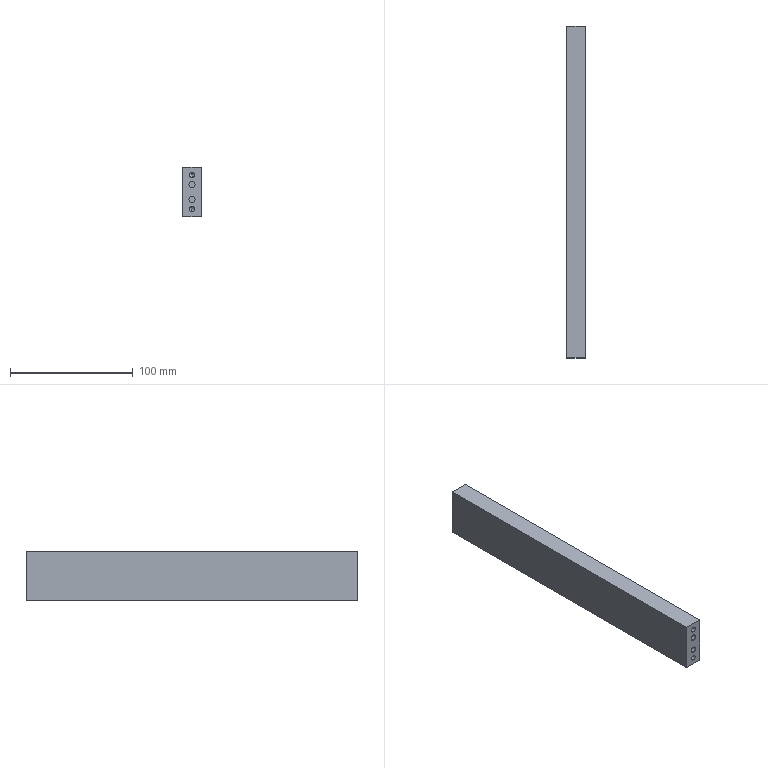Component | SolidWorks | PressingMechanism-12-2 | 1 solid | 34 faces | box 15 x 270 x 40 mm | volume 160573 mm3 | cylinder 16 | plane 10 | cone 8 | commonest cylinder face diameters 5 x8 4.2 x8
build123d program:
from build123d import *

# Parameters (mm, degrees)
SKETCH1_W             = 270
SKETCH1_H             = 40
EXTRUDE1_DEPTH        = 7.5
M5_TAPPED_HOLE1_D     = 4.2
M5_TAPPED_HOLE1_DEPTH = 14
M5_TAPPED_HOLE1_TIP   = 1.262
M5_TAPPED_HOLE2_D     = 4.2
M5_TAPPED_HOLE2_DEPTH = 14
M5_TAPPED_HOLE2_TIP   = 1.262
HOLEWZD1_D            = 5
HOLEWZD1_DEPTH        = 8
HOLEWZD2_D            = 5
HOLEWZD2_DEPTH        = 8


with BuildPart() as part:
    # Sketch1 → Extrude1 (new, symmetric)
    with BuildSketch(Plane(origin=(0, 0, 0), x_dir=(1, 0, 0), z_dir=(0, 1, 0))):
        Rectangle(SKETCH1_W, SKETCH1_H)
    extrude(amount=EXTRUDE1_DEPTH, both=True)

    # M5 Tapped Hole1
    with Locations(Plane(origin=(135, 0, 0), x_dir=(0, 0, -1), z_dir=(1, 0, 0))):
        with Locations((14, 0), (-14, 0)):
            Hole(M5_TAPPED_HOLE1_D / 2, depth=M5_TAPPED_HOLE1_DEPTH)
            with Locations((0, 0, -(M5_TAPPED_HOLE1_DEPTH + M5_TAPPED_HOLE1_TIP / 2))):  # 118° drill point
                Cone(0, M5_TAPPED_HOLE1_D / 2, M5_TAPPED_HOLE1_TIP, mode=Mode.SUBTRACT)

    # M5 Tapped Hole2
    with Locations(Plane.ZY.offset(135)):
        with Locations((-14, 0), (14, 0)):
            Hole(M5_TAPPED_HOLE2_D / 2, depth=M5_TAPPED_HOLE2_DEPTH)
            with Locations((0, 0, -(M5_TAPPED_HOLE2_DEPTH + M5_TAPPED_HOLE2_TIP / 2))):  # 118° drill point
                Cone(0, M5_TAPPED_HOLE2_D / 2, M5_TAPPED_HOLE2_TIP, mode=Mode.SUBTRACT)

    # HoleWzd1
    with Locations(Plane(origin=(135, 0, 0), x_dir=(0, 0, -1), z_dir=(1, 0, 0))):
        with Locations((6, 0), (-6, 0)):
            Hole(HOLEWZD1_D / 2, depth=HOLEWZD1_DEPTH)

    # HoleWzd2
    with Locations(Plane.ZY.offset(135)):
        with Locations((-6, 0), (6, 0)):
            Hole(HOLEWZD2_D / 2, depth=HOLEWZD2_DEPTH)


solid = part.part

# Placed as in the assembly
solid = solid.moved(Location((-192.5, -90, 77), (0, 0, 90)))
STEP:
#1=CARTESIAN_POINT('',(-7.579,-8.543,3.366));
#2=VERTEX_POINT('',#1);
#3=CARTESIAN_POINT('',(-7.579,-8.543,3.169));
#4=VERTEX_POINT('',#3);
#5=CARTESIAN_POINT('',(-7.579,-8.543,3.268));
#6=DIRECTION('',(0.,-1.,0.));
#7=DIRECTION('',(0.,0.,-1.));
#8=AXIS2_PLACEMENT_3D('',#5,#6,#7);
#9=CIRCLE('',#8,0.09843);
#10=EDGE_CURVE('',#2,#4,#9,.T.);
#11=ORIENTED_EDGE('',*,*,#10,.F.);
#12=CARTESIAN_POINT('',(-7.579,-8.858,3.366));
#13=VERTEX_POINT('',#12);
#14=CARTESIAN_POINT('',(-7.579,-8.858,3.366));
#15=DIRECTION('',(0.,-1.,0.));
#16=VECTOR('',#15,39.37);
#17=LINE('',#14,#16);
#18=EDGE_CURVE('',#2,#13,#17,.T.);
#19=ORIENTED_EDGE('',*,*,#18,.T.);
#20=CARTESIAN_POINT('',(-7.579,-8.858,3.169));
#21=VERTEX_POINT('',#20);
#22=CARTESIAN_POINT('',(-7.579,-8.858,3.268));
#23=DIRECTION('',(0.,-1.,0.));
#24=DIRECTION('',(0.,0.,-1.));
#25=AXIS2_PLACEMENT_3D('',#22,#23,#24);
#26=CIRCLE('',#25,0.09843);
#27=EDGE_CURVE('',#13,#21,#26,.T.);
#28=ORIENTED_EDGE('',*,*,#27,.T.);
#29=CARTESIAN_POINT('',(-7.579,-8.858,3.169));
#30=DIRECTION('',(0.,-1.,0.));
#31=VECTOR('',#30,39.37);
#32=LINE('',#29,#31);
#33=EDGE_CURVE('',#4,#21,#32,.T.);
#34=ORIENTED_EDGE('',*,*,#33,.F.);
#35=EDGE_LOOP('',(#11,#19,#28,#34));
#36=FACE_OUTER_BOUND('',#35,.T.);
#37=CARTESIAN_POINT('',(-7.579,-8.858,3.268));
#38=DIRECTION('',(0.,-1.,0.));
#39=DIRECTION('',(0.,0.,-1.));
#40=AXIS2_PLACEMENT_3D('',#37,#38,#39);
#41=CYLINDRICAL_SURFACE('',#40,0.09843);
#42=ADVANCED_FACE('',(#36),#41,.F.);
#43=CARTESIAN_POINT('',(-7.579,-8.543,2.894));
#44=VERTEX_POINT('',#43);
#45=CARTESIAN_POINT('',(-7.579,-8.543,2.697));
#46=VERTEX_POINT('',#45);
#47=CARTESIAN_POINT('',(-7.579,-8.543,2.795));
#48=DIRECTION('',(0.,-1.,0.));
#49=DIRECTION('',(0.,0.,-1.));
#50=AXIS2_PLACEMENT_3D('',#47,#48,#49);
#51=CIRCLE('',#50,0.09843);
#52=EDGE_CURVE('',#44,#46,#51,.T.);
#53=ORIENTED_EDGE('',*,*,#52,.F.);
#54=CARTESIAN_POINT('',(-7.579,-8.858,2.894));
#55=VERTEX_POINT('',#54);
#56=CARTESIAN_POINT('',(-7.579,-8.858,2.894));
#57=DIRECTION('',(0.,-1.,0.));
#58=VECTOR('',#57,39.37);
#59=LINE('',#56,#58);
#60=EDGE_CURVE('',#44,#55,#59,.T.);
#61=ORIENTED_EDGE('',*,*,#60,.T.);
#62=CARTESIAN_POINT('',(-7.579,-8.858,2.697));
#63=VERTEX_POINT('',#62);
#64=CARTESIAN_POINT('',(-7.579,-8.858,2.795));
#65=DIRECTION('',(0.,-1.,0.));
#66=DIRECTION('',(0.,0.,-1.));
#67=AXIS2_PLACEMENT_3D('',#64,#65,#66);
#68=CIRCLE('',#67,0.09843);
#69=EDGE_CURVE('',#55,#63,#68,.T.);
#70=ORIENTED_EDGE('',*,*,#69,.T.);
#71=CARTESIAN_POINT('',(-7.579,-8.858,2.697));
#72=DIRECTION('',(0.,-1.,0.));
#73=VECTOR('',#72,39.37);
#74=LINE('',#71,#73);
#75=EDGE_CURVE('',#46,#63,#74,.T.);
#76=ORIENTED_EDGE('',*,*,#75,.F.);
#77=EDGE_LOOP('',(#53,#61,#70,#76));
#78=FACE_OUTER_BOUND('',#77,.T.);
#79=CARTESIAN_POINT('',(-7.579,-8.858,2.795));
#80=DIRECTION('',(0.,-1.,0.));
#81=DIRECTION('',(0.,0.,-1.));
#82=AXIS2_PLACEMENT_3D('',#79,#80,#81);
#83=CYLINDRICAL_SURFACE('',#82,0.09843);
#84=ADVANCED_FACE('',(#78),#83,.F.);
#85=CARTESIAN_POINT('',(-7.579,1.457,3.169));
#86=VERTEX_POINT('',#85);
#87=CARTESIAN_POINT('',(-7.579,1.457,3.366));
#88=VERTEX_POINT('',#87);
#89=CARTESIAN_POINT('',(-7.579,1.457,3.268));
#90=DIRECTION('',(-0.,1.,-0.));
#91=DIRECTION('',(0.,0.,1.));
#92=AXIS2_PLACEMENT_3D('',#89,#90,#91);
#93=CIRCLE('',#92,0.09843);
#94=EDGE_CURVE('',#86,#88,#93,.T.);
#95=ORIENTED_EDGE('',*,*,#94,.F.);
#96=CARTESIAN_POINT('',(-7.579,1.772,3.169));
#97=VERTEX_POINT('',#96);
#98=CARTESIAN_POINT('',(-7.579,1.772,3.169));
#99=DIRECTION('',(-0.,1.,-0.));
#100=VECTOR('',#99,39.37);
#101=LINE('',#98,#100);
#102=EDGE_CURVE('',#86,#97,#101,.T.);
#103=ORIENTED_EDGE('',*,*,#102,.T.);
#104=CARTESIAN_POINT('',(-7.579,1.772,3.366));
#105=VERTEX_POINT('',#104);
#106=CARTESIAN_POINT('',(-7.579,1.772,3.268));
#107=DIRECTION('',(-0.,1.,-0.));
#108=DIRECTION('',(0.,0.,1.));
#109=AXIS2_PLACEMENT_3D('',#106,#107,#108);
#110=CIRCLE('',#109,0.09843);
#111=EDGE_CURVE('',#97,#105,#110,.T.);
#112=ORIENTED_EDGE('',*,*,#111,.T.);
#113=CARTESIAN_POINT('',(-7.579,1.772,3.366));
#114=DIRECTION('',(-0.,1.,-0.));
#115=VECTOR('',#114,39.37);
#116=LINE('',#113,#115);
#117=EDGE_CURVE('',#88,#105,#116,.T.);
#118=ORIENTED_EDGE('',*,*,#117,.F.);
#119=EDGE_LOOP('',(#95,#103,#112,#118));
#120=FACE_OUTER_BOUND('',#119,.T.);
#121=CARTESIAN_POINT('',(-7.579,1.772,3.268));
#122=DIRECTION('',(-0.,1.,-0.));
#123=DIRECTION('',(0.,0.,1.));
#124=AXIS2_PLACEMENT_3D('',#121,#122,#123);
#125=CYLINDRICAL_SURFACE('',#124,0.09843);
#126=ADVANCED_FACE('',(#120),#125,.F.);
#127=CARTESIAN_POINT('',(-7.579,1.457,2.697));
#128=VERTEX_POINT('',#127);
#129=CARTESIAN_POINT('',(-7.579,1.457,2.894));
#130=VERTEX_POINT('',#129);
#131=CARTESIAN_POINT('',(-7.579,1.457,2.795));
#132=DIRECTION('',(-0.,1.,-0.));
#133=DIRECTION('',(0.,0.,1.));
#134=AXIS2_PLACEMENT_3D('',#131,#132,#133);
#135=CIRCLE('',#134,0.09843);
#136=EDGE_CURVE('',#128,#130,#135,.T.);
#137=ORIENTED_EDGE('',*,*,#136,.F.);
#138=CARTESIAN_POINT('',(-7.579,1.772,2.697));
#139=VERTEX_POINT('',#138);
#140=CARTESIAN_POINT('',(-7.579,1.772,2.697));
#141=DIRECTION('',(-0.,1.,-0.));
#142=VECTOR('',#141,39.37);
#143=LINE('',#140,#142);
#144=EDGE_CURVE('',#128,#139,#143,.T.);
#145=ORIENTED_EDGE('',*,*,#144,.T.);
#146=CARTESIAN_POINT('',(-7.579,1.772,2.894));
#147=VERTEX_POINT('',#146);
#148=CARTESIAN_POINT('',(-7.579,1.772,2.795));
#149=DIRECTION('',(-0.,1.,-0.));
#150=DIRECTION('',(0.,0.,1.));
#151=AXIS2_PLACEMENT_3D('',#148,#149,#150);
#152=CIRCLE('',#151,0.09843);
#153=EDGE_CURVE('',#139,#147,#152,.T.);
#154=ORIENTED_EDGE('',*,*,#153,.T.);
#155=CARTESIAN_POINT('',(-7.579,1.772,2.894));
#156=DIRECTION('',(-0.,1.,-0.));
#157=VECTOR('',#156,39.37);
#158=LINE('',#155,#157);
#159=EDGE_CURVE('',#130,#147,#158,.T.);
#160=ORIENTED_EDGE('',*,*,#159,.F.);
#161=EDGE_LOOP('',(#137,#145,#154,#160));
#162=FACE_OUTER_BOUND('',#161,.T.);
#163=CARTESIAN_POINT('',(-7.579,1.772,2.795));
#164=DIRECTION('',(-0.,1.,-0.));
#165=DIRECTION('',(0.,0.,1.));
#166=AXIS2_PLACEMENT_3D('',#163,#164,#165);
#167=CYLINDRICAL_SURFACE('',#166,0.09843);
#168=ADVANCED_FACE('',(#162),#167,.F.);
#169=CARTESIAN_POINT('',(-7.579,-8.307,3.665));
#170=VERTEX_POINT('',#169);
#171=CARTESIAN_POINT('',(-7.579,-8.307,3.5));
#172=VERTEX_POINT('',#171);
#173=CARTESIAN_POINT('',(-7.579,-8.307,3.583));
#174=DIRECTION('',(0.,-1.,0.));
#175=DIRECTION('',(0.,0.,-1.));
#176=AXIS2_PLACEMENT_3D('',#173,#174,#175);
#177=CIRCLE('',#176,0.08268);
#178=EDGE_CURVE('',#170,#172,#177,.T.);
#179=ORIENTED_EDGE('',*,*,#178,.F.);
#180=CARTESIAN_POINT('',(-7.579,-8.858,3.665));
#181=VERTEX_POINT('',#180);
#182=CARTESIAN_POINT('',(-7.579,-8.858,3.665));
#183=DIRECTION('',(0.,-1.,0.));
#184=VECTOR('',#183,39.37);
#185=LINE('',#182,#184);
#186=EDGE_CURVE('',#170,#181,#185,.T.);
#187=ORIENTED_EDGE('',*,*,#186,.T.);
#188=CARTESIAN_POINT('',(-7.579,-8.858,3.5));
#189=VERTEX_POINT('',#188);
#190=CARTESIAN_POINT('',(-7.579,-8.858,3.583));
#191=DIRECTION('',(0.,-1.,0.));
#192=DIRECTION('',(0.,0.,-1.));
#193=AXIS2_PLACEMENT_3D('',#190,#191,#192);
#194=CIRCLE('',#193,0.08268);
#195=EDGE_CURVE('',#181,#189,#194,.T.);
#196=ORIENTED_EDGE('',*,*,#195,.T.);
#197=CARTESIAN_POINT('',(-7.579,-8.858,3.5));
#198=DIRECTION('',(0.,-1.,0.));
#199=VECTOR('',#198,39.37);
#200=LINE('',#197,#199);
#201=EDGE_CURVE('',#172,#189,#200,.T.);
#202=ORIENTED_EDGE('',*,*,#201,.F.);
#203=EDGE_LOOP('',(#179,#187,#196,#202));
#204=FACE_OUTER_BOUND('',#203,.T.);
#205=CARTESIAN_POINT('',(-7.579,-8.858,3.583));
#206=DIRECTION('',(0.,-1.,0.));
#207=DIRECTION('',(0.,0.,-1.));
#208=AXIS2_PLACEMENT_3D('',#205,#206,#207);
#209=CYLINDRICAL_SURFACE('',#208,0.08268);
#210=ADVANCED_FACE('',(#204),#209,.F.);
#211=CARTESIAN_POINT('',(-7.579,-8.257,3.583));
#212=VERTEX_POINT('',#211);
#213=CARTESIAN_POINT('',(-7.579,-8.307,3.5));
#214=DIRECTION('',(-0.,-0.515,-0.8572));
#215=VECTOR('',#214,39.37);
#216=LINE('',#213,#215);
#217=EDGE_CURVE('',#212,#172,#216,.T.);
#218=ORIENTED_EDGE('',*,*,#217,.F.);
#219=CARTESIAN_POINT('',(-7.579,-8.307,3.665));
#220=DIRECTION('',(0.,-0.515,0.8572));
#221=VECTOR('',#220,39.37);
#222=LINE('',#219,#221);
#223=EDGE_CURVE('',#212,#170,#222,.T.);
#224=ORIENTED_EDGE('',*,*,#223,.T.);
#225=ORIENTED_EDGE('',*,*,#178,.T.);
#226=EDGE_LOOP('',(#218,#224,#225));
#227=FACE_OUTER_BOUND('',#226,.T.);
#228=CARTESIAN_POINT('',(-7.579,-8.307,3.583));
#229=DIRECTION('',(0.,-1.,0.));
#230=DIRECTION('',(0.,0.,-1.));
#231=AXIS2_PLACEMENT_3D('',#228,#229,#230);
#232=CONICAL_SURFACE('',#231,0.08268,1.03);
#233=ADVANCED_FACE('',(#227),#232,.F.);
#234=CARTESIAN_POINT('',(-7.579,-8.307,2.563));
#235=VERTEX_POINT('',#234);
#236=CARTESIAN_POINT('',(-7.579,-8.307,2.398));
#237=VERTEX_POINT('',#236);
#238=CARTESIAN_POINT('',(-7.579,-8.307,2.48));
#239=DIRECTION('',(0.,-1.,0.));
#240=DIRECTION('',(0.,0.,-1.));
#241=AXIS2_PLACEMENT_3D('',#238,#239,#240);
#242=CIRCLE('',#241,0.08268);
#243=EDGE_CURVE('',#235,#237,#242,.T.);
#244=ORIENTED_EDGE('',*,*,#243,.F.);
#245=CARTESIAN_POINT('',(-7.579,-8.858,2.563));
#246=VERTEX_POINT('',#245);
#247=CARTESIAN_POINT('',(-7.579,-8.858,2.563));
#248=DIRECTION('',(0.,-1.,0.));
#249=VECTOR('',#248,39.37);
#250=LINE('',#247,#249);
#251=EDGE_CURVE('',#235,#246,#250,.T.);
#252=ORIENTED_EDGE('',*,*,#251,.T.);
#253=CARTESIAN_POINT('',(-7.579,-8.858,2.398));
#254=VERTEX_POINT('',#253);
#255=CARTESIAN_POINT('',(-7.579,-8.858,2.48));
#256=DIRECTION('',(0.,-1.,0.));
#257=DIRECTION('',(0.,0.,-1.));
#258=AXIS2_PLACEMENT_3D('',#255,#256,#257);
#259=CIRCLE('',#258,0.08268);
#260=EDGE_CURVE('',#246,#254,#259,.T.);
#261=ORIENTED_EDGE('',*,*,#260,.T.);
#262=CARTESIAN_POINT('',(-7.579,-8.858,2.398));
#263=DIRECTION('',(0.,-1.,0.));
#264=VECTOR('',#263,39.37);
#265=LINE('',#262,#264);
#266=EDGE_CURVE('',#237,#254,#265,.T.);
#267=ORIENTED_EDGE('',*,*,#266,.F.);
#268=EDGE_LOOP('',(#244,#252,#261,#267));
#269=FACE_OUTER_BOUND('',#268,.T.);
#270=CARTESIAN_POINT('',(-7.579,-8.858,2.48));
#271=DIRECTION('',(0.,-1.,0.));
#272=DIRECTION('',(0.,0.,-1.));
#273=AXIS2_PLACEMENT_3D('',#270,#271,#272);
#274=CYLINDRICAL_SURFACE('',#273,0.08268);
#275=ADVANCED_FACE('',(#269),#274,.F.);
#276=CARTESIAN_POINT('',(-7.579,-8.257,2.48));
#277=VERTEX_POINT('',#276);
#278=CARTESIAN_POINT('',(-7.579,-8.307,2.398));
#279=DIRECTION('',(-0.,-0.515,-0.8572));
#280=VECTOR('',#279,39.37);
#281=LINE('',#278,#280);
#282=EDGE_CURVE('',#277,#237,#281,.T.);
#283=ORIENTED_EDGE('',*,*,#282,.F.);
#284=CARTESIAN_POINT('',(-7.579,-8.307,2.563));
#285=DIRECTION('',(0.,-0.515,0.8572));
#286=VECTOR('',#285,39.37);
#287=LINE('',#284,#286);
#288=EDGE_CURVE('',#277,#235,#287,.T.);
#289=ORIENTED_EDGE('',*,*,#288,.T.);
#290=ORIENTED_EDGE('',*,*,#243,.T.);
#291=EDGE_LOOP('',(#283,#289,#290));
#292=FACE_OUTER_BOUND('',#291,.T.);
#293=CARTESIAN_POINT('',(-7.579,-8.307,2.48));
#294=DIRECTION('',(0.,-1.,0.));
#295=DIRECTION('',(0.,0.,-1.));
#296=AXIS2_PLACEMENT_3D('',#293,#294,#295);
#297=CONICAL_SURFACE('',#296,0.08268,1.03);
#298=ADVANCED_FACE('',(#292),#297,.F.);
#299=CARTESIAN_POINT('',(-7.579,1.22,3.5));
#300=VERTEX_POINT('',#299);
#301=CARTESIAN_POINT('',(-7.579,1.22,3.665));
#302=VERTEX_POINT('',#301);
#303=CARTESIAN_POINT('',(-7.579,1.22,3.583));
#304=DIRECTION('',(-0.,1.,-0.));
#305=DIRECTION('',(0.,0.,1.));
#306=AXIS2_PLACEMENT_3D('',#303,#304,#305);
#307=CIRCLE('',#306,0.08268);
#308=EDGE_CURVE('',#300,#302,#307,.T.);
#309=ORIENTED_EDGE('',*,*,#308,.F.);
#310=CARTESIAN_POINT('',(-7.579,1.772,3.5));
#311=VERTEX_POINT('',#310);
#312=CARTESIAN_POINT('',(-7.579,1.772,3.5));
#313=DIRECTION('',(-0.,1.,-0.));
#314=VECTOR('',#313,39.37);
#315=LINE('',#312,#314);
#316=EDGE_CURVE('',#300,#311,#315,.T.);
#317=ORIENTED_EDGE('',*,*,#316,.T.);
#318=CARTESIAN_POINT('',(-7.579,1.772,3.665));
#319=VERTEX_POINT('',#318);
#320=CARTESIAN_POINT('',(-7.579,1.772,3.583));
#321=DIRECTION('',(-0.,1.,-0.));
#322=DIRECTION('',(0.,0.,1.));
#323=AXIS2_PLACEMENT_3D('',#320,#321,#322);
#324=CIRCLE('',#323,0.08268);
#325=EDGE_CURVE('',#311,#319,#324,.T.);
#326=ORIENTED_EDGE('',*,*,#325,.T.);
#327=CARTESIAN_POINT('',(-7.579,1.772,3.665));
#328=DIRECTION('',(-0.,1.,-0.));
#329=VECTOR('',#328,39.37);
#330=LINE('',#327,#329);
#331=EDGE_CURVE('',#302,#319,#330,.T.);
#332=ORIENTED_EDGE('',*,*,#331,.F.);
#333=EDGE_LOOP('',(#309,#317,#326,#332));
#334=FACE_OUTER_BOUND('',#333,.T.);
#335=CARTESIAN_POINT('',(-7.579,1.772,3.583));
#336=DIRECTION('',(-0.,1.,-0.));
#337=DIRECTION('',(0.,0.,1.));
#338=AXIS2_PLACEMENT_3D('',#335,#336,#337);
#339=CYLINDRICAL_SURFACE('',#338,0.08268);
#340=ADVANCED_FACE('',(#334),#339,.F.);
#341=CARTESIAN_POINT('',(-7.579,1.171,3.583));
#342=VERTEX_POINT('',#341);
#343=CARTESIAN_POINT('',(-7.579,1.22,3.665));
#344=DIRECTION('',(0.,0.515,0.8572));
#345=VECTOR('',#344,39.37);
#346=LINE('',#343,#345);
#347=EDGE_CURVE('',#342,#302,#346,.T.);
#348=ORIENTED_EDGE('',*,*,#347,.F.);
#349=CARTESIAN_POINT('',(-7.579,1.22,3.5));
#350=DIRECTION('',(-0.,0.515,-0.8572));
#351=VECTOR('',#350,39.37);
#352=LINE('',#349,#351);
#353=EDGE_CURVE('',#342,#300,#352,.T.);
#354=ORIENTED_EDGE('',*,*,#353,.T.);
#355=ORIENTED_EDGE('',*,*,#308,.T.);
#356=EDGE_LOOP('',(#348,#354,#355));
#357=FACE_OUTER_BOUND('',#356,.T.);
#358=CARTESIAN_POINT('',(-7.579,1.22,3.583));
#359=DIRECTION('',(-0.,1.,-0.));
#360=DIRECTION('',(0.,0.,1.));
#361=AXIS2_PLACEMENT_3D('',#358,#359,#360);
#362=CONICAL_SURFACE('',#361,0.08268,1.03);
#363=ADVANCED_FACE('',(#357),#362,.F.);
#364=CARTESIAN_POINT('',(-7.579,1.22,2.398));
#365=VERTEX_POINT('',#364);
#366=CARTESIAN_POINT('',(-7.579,1.22,2.563));
#367=VERTEX_POINT('',#366);
#368=CARTESIAN_POINT('',(-7.579,1.22,2.48));
#369=DIRECTION('',(-0.,1.,-0.));
#370=DIRECTION('',(0.,0.,1.));
#371=AXIS2_PLACEMENT_3D('',#368,#369,#370);
#372=CIRCLE('',#371,0.08268);
#373=EDGE_CURVE('',#365,#367,#372,.T.);
#374=ORIENTED_EDGE('',*,*,#373,.F.);
#375=CARTESIAN_POINT('',(-7.579,1.772,2.398));
#376=VERTEX_POINT('',#375);
#377=CARTESIAN_POINT('',(-7.579,1.772,2.398));
#378=DIRECTION('',(-0.,1.,-0.));
#379=VECTOR('',#378,39.37);
#380=LINE('',#377,#379);
#381=EDGE_CURVE('',#365,#376,#380,.T.);
#382=ORIENTED_EDGE('',*,*,#381,.T.);
#383=CARTESIAN_POINT('',(-7.579,1.772,2.563));
#384=VERTEX_POINT('',#383);
#385=CARTESIAN_POINT('',(-7.579,1.772,2.48));
#386=DIRECTION('',(-0.,1.,-0.));
#387=DIRECTION('',(0.,0.,1.));
#388=AXIS2_PLACEMENT_3D('',#385,#386,#387);
#389=CIRCLE('',#388,0.08268);
#390=EDGE_CURVE('',#376,#384,#389,.T.);
#391=ORIENTED_EDGE('',*,*,#390,.T.);
#392=CARTESIAN_POINT('',(-7.579,1.772,2.563));
#393=DIRECTION('',(-0.,1.,-0.));
#394=VECTOR('',#393,39.37);
#395=LINE('',#392,#394);
#396=EDGE_CURVE('',#367,#384,#395,.T.);
#397=ORIENTED_EDGE('',*,*,#396,.F.);
#398=EDGE_LOOP('',(#374,#382,#391,#397));
#399=FACE_OUTER_BOUND('',#398,.T.);
#400=CARTESIAN_POINT('',(-7.579,1.772,2.48));
#401=DIRECTION('',(-0.,1.,-0.));
#402=DIRECTION('',(0.,0.,1.));
#403=AXIS2_PLACEMENT_3D('',#400,#401,#402);
#404=CYLINDRICAL_SURFACE('',#403,0.08268);
#405=ADVANCED_FACE('',(#399),#404,.F.);
#406=CARTESIAN_POINT('',(-7.579,1.171,2.48));
#407=VERTEX_POINT('',#406);
#408=CARTESIAN_POINT('',(-7.579,1.22,2.563));
#409=DIRECTION('',(0.,0.515,0.8572));
#410=VECTOR('',#409,39.37);
#411=LINE('',#408,#410);
#412=EDGE_CURVE('',#407,#367,#411,.T.);
#413=ORIENTED_EDGE('',*,*,#412,.F.);
#414=CARTESIAN_POINT('',(-7.579,1.22,2.398));
#415=DIRECTION('',(-0.,0.515,-0.8572));
#416=VECTOR('',#415,39.37);
#417=LINE('',#414,#416);
#418=EDGE_CURVE('',#407,#365,#417,.T.);
#419=ORIENTED_EDGE('',*,*,#418,.T.);
#420=ORIENTED_EDGE('',*,*,#373,.T.);
#421=EDGE_LOOP('',(#413,#419,#420));
#422=FACE_OUTER_BOUND('',#421,.T.);
#423=CARTESIAN_POINT('',(-7.579,1.22,2.48));
#424=DIRECTION('',(-0.,1.,-0.));
#425=DIRECTION('',(0.,0.,1.));
#426=AXIS2_PLACEMENT_3D('',#423,#424,#425);
#427=CONICAL_SURFACE('',#426,0.08268,1.03);
#428=ADVANCED_FACE('',(#422),#427,.F.);
#429=CARTESIAN_POINT('',(-7.579,-8.858,3.268));
#430=DIRECTION('',(0.,-1.,0.));
#431=DIRECTION('',(0.,0.,-1.));
#432=AXIS2_PLACEMENT_3D('',#429,#430,#431);
#433=CIRCLE('',#432,0.09843);
#434=EDGE_CURVE('',#21,#13,#433,.T.);
#435=ORIENTED_EDGE('',*,*,#434,.F.);
#436=ORIENTED_EDGE('',*,*,#27,.F.);
#437=EDGE_LOOP('',(#435,#436));
#438=FACE_BOUND('',#437,.T.);
#439=CARTESIAN_POINT('',(-7.579,-8.858,2.795));
#440=DIRECTION('',(0.,-1.,0.));
#441=DIRECTION('',(0.,0.,-1.));
#442=AXIS2_PLACEMENT_3D('',#439,#440,#441);
#443=CIRCLE('',#442,0.09843);
#444=EDGE_CURVE('',#63,#55,#443,.T.);
#445=ORIENTED_EDGE('',*,*,#444,.F.);
#446=ORIENTED_EDGE('',*,*,#69,.F.);
#447=EDGE_LOOP('',(#445,#446));
#448=FACE_BOUND('',#447,.T.);
#449=CARTESIAN_POINT('',(-7.579,-8.858,3.583));
#450=DIRECTION('',(0.,-1.,0.));
#451=DIRECTION('',(0.,0.,-1.));
#452=AXIS2_PLACEMENT_3D('',#449,#450,#451);
#453=CIRCLE('',#452,0.08268);
#454=EDGE_CURVE('',#189,#181,#453,.T.);
#455=ORIENTED_EDGE('',*,*,#454,.F.);
#456=ORIENTED_EDGE('',*,*,#195,.F.);
#457=EDGE_LOOP('',(#455,#456));
#458=FACE_BOUND('',#457,.T.);
#459=CARTESIAN_POINT('',(-7.579,-8.858,2.48));
#460=DIRECTION('',(0.,-1.,0.));
#461=DIRECTION('',(0.,0.,-1.));
#462=AXIS2_PLACEMENT_3D('',#459,#460,#461);
#463=CIRCLE('',#462,0.08268);
#464=EDGE_CURVE('',#254,#246,#463,.T.);
#465=ORIENTED_EDGE('',*,*,#464,.F.);
#466=ORIENTED_EDGE('',*,*,#260,.F.);
#467=EDGE_LOOP('',(#465,#466));
#468=FACE_BOUND('',#467,.T.);
#469=CARTESIAN_POINT('',(-7.874,-8.858,3.819));
#470=VERTEX_POINT('',#469);
#471=CARTESIAN_POINT('',(-7.874,-8.858,2.244));
#472=VERTEX_POINT('',#471);
#473=CARTESIAN_POINT('',(-7.874,-8.858,3.819));
#474=DIRECTION('',(-0.,-0.,-1.));
#475=VECTOR('',#474,39.37);
#476=LINE('',#473,#475);
#477=EDGE_CURVE('',#470,#472,#476,.T.);
#478=ORIENTED_EDGE('',*,*,#477,.T.);
#479=CARTESIAN_POINT('',(-7.283,-8.858,2.244));
#480=VERTEX_POINT('',#479);
#481=CARTESIAN_POINT('',(-7.283,-8.858,2.244));
#482=DIRECTION('',(-1.,0.,0.));
#483=VECTOR('',#482,39.37);
#484=LINE('',#481,#483);
#485=EDGE_CURVE('',#480,#472,#484,.T.);
#486=ORIENTED_EDGE('',*,*,#485,.F.);
#487=CARTESIAN_POINT('',(-7.283,-8.858,3.819));
#488=VERTEX_POINT('',#487);
#489=CARTESIAN_POINT('',(-7.283,-8.858,3.819));
#490=DIRECTION('',(-0.,-0.,-1.));
#491=VECTOR('',#490,39.37);
#492=LINE('',#489,#491);
#493=EDGE_CURVE('',#488,#480,#492,.T.);
#494=ORIENTED_EDGE('',*,*,#493,.F.);
#495=CARTESIAN_POINT('',(-7.283,-8.858,3.819));
#496=DIRECTION('',(-1.,0.,0.));
#497=VECTOR('',#496,39.37);
#498=LINE('',#495,#497);
#499=EDGE_CURVE('',#488,#470,#498,.T.);
#500=ORIENTED_EDGE('',*,*,#499,.T.);
#501=EDGE_LOOP('',(#478,#486,#494,#500));
#502=FACE_OUTER_BOUND('',#501,.T.);
#503=CARTESIAN_POINT('',(-7.283,-8.858,3.819));
#504=DIRECTION('',(-0.,1.,-0.));
#505=DIRECTION('',(0.,0.,1.));
#506=AXIS2_PLACEMENT_3D('',#503,#504,#505);
#507=PLANE('',#506);
#508=ADVANCED_FACE('',(#438,#448,#458,#468,#502),#507,.F.);
#509=CARTESIAN_POINT('',(-7.874,1.772,2.244));
#510=VERTEX_POINT('',#509);
#511=CARTESIAN_POINT('',(-7.874,-8.858,2.244));
#512=DIRECTION('',(-0.,1.,-0.));
#513=VECTOR('',#512,39.37);
#514=LINE('',#511,#513);
#515=EDGE_CURVE('',#472,#510,#514,.T.);
#516=ORIENTED_EDGE('',*,*,#515,.T.);
#517=CARTESIAN_POINT('',(-7.283,1.772,2.244));
#518=VERTEX_POINT('',#517);
#519=CARTESIAN_POINT('',(-7.283,1.772,2.244));
#520=DIRECTION('',(-1.,0.,0.));
#521=VECTOR('',#520,39.37);
#522=LINE('',#519,#521);
#523=EDGE_CURVE('',#518,#510,#522,.T.);
#524=ORIENTED_EDGE('',*,*,#523,.F.);
#525=CARTESIAN_POINT('',(-7.283,-8.858,2.244));
#526=DIRECTION('',(-0.,1.,-0.));
#527=VECTOR('',#526,39.37);
#528=LINE('',#525,#527);
#529=EDGE_CURVE('',#480,#518,#528,.T.);
#530=ORIENTED_EDGE('',*,*,#529,.F.);
#531=ORIENTED_EDGE('',*,*,#485,.T.);
#532=EDGE_LOOP('',(#516,#524,#530,#531));
#533=FACE_OUTER_BOUND('',#532,.T.);
#534=CARTESIAN_POINT('',(-7.283,-8.858,2.244));
#535=DIRECTION('',(0.,0.,1.));
#536=DIRECTION('',(0.,-1.,0.));
#537=AXIS2_PLACEMENT_3D('',#534,#535,#536);
#538=PLANE('',#537);
#539=ADVANCED_FACE('',(#533),#538,.F.);
#540=CARTESIAN_POINT('',(-7.579,1.772,3.268));
#541=DIRECTION('',(-0.,1.,-0.));
#542=DIRECTION('',(0.,0.,1.));
#543=AXIS2_PLACEMENT_3D('',#540,#541,#542);
#544=CIRCLE('',#543,0.09843);
#545=EDGE_CURVE('',#105,#97,#544,.T.);
#546=ORIENTED_EDGE('',*,*,#545,.F.);
#547=ORIENTED_EDGE('',*,*,#111,.F.);
#548=EDGE_LOOP('',(#546,#547));
#549=FACE_BOUND('',#548,.T.);
#550=CARTESIAN_POINT('',(-7.579,1.772,2.795));
#551=DIRECTION('',(-0.,1.,-0.));
#552=DIRECTION('',(0.,0.,1.));
#553=AXIS2_PLACEMENT_3D('',#550,#551,#552);
#554=CIRCLE('',#553,0.09843);
#555=EDGE_CURVE('',#147,#139,#554,.T.);
#556=ORIENTED_EDGE('',*,*,#555,.F.);
#557=ORIENTED_EDGE('',*,*,#153,.F.);
#558=EDGE_LOOP('',(#556,#557));
#559=FACE_BOUND('',#558,.T.);
#560=CARTESIAN_POINT('',(-7.579,1.772,3.583));
#561=DIRECTION('',(-0.,1.,-0.));
#562=DIRECTION('',(0.,0.,1.));
#563=AXIS2_PLACEMENT_3D('',#560,#561,#562);
#564=CIRCLE('',#563,0.08268);
#565=EDGE_CURVE('',#319,#311,#564,.T.);
#566=ORIENTED_EDGE('',*,*,#565,.F.);
#567=ORIENTED_EDGE('',*,*,#325,.F.);
#568=EDGE_LOOP('',(#566,#567));
#569=FACE_BOUND('',#568,.T.);
#570=CARTESIAN_POINT('',(-7.579,1.772,2.48));
#571=DIRECTION('',(-0.,1.,-0.));
#572=DIRECTION('',(0.,0.,1.));
#573=AXIS2_PLACEMENT_3D('',#570,#571,#572);
#574=CIRCLE('',#573,0.08268);
#575=EDGE_CURVE('',#384,#376,#574,.T.);
#576=ORIENTED_EDGE('',*,*,#575,.F.);
#577=ORIENTED_EDGE('',*,*,#390,.F.);
#578=EDGE_LOOP('',(#576,#577));
#579=FACE_BOUND('',#578,.T.);
#580=CARTESIAN_POINT('',(-7.874,1.772,3.819));
#581=VERTEX_POINT('',#580);
#582=CARTESIAN_POINT('',(-7.874,1.772,3.819));
#583=DIRECTION('',(0.,0.,1.));
#584=VECTOR('',#583,39.37);
#585=LINE('',#582,#584);
#586=EDGE_CURVE('',#510,#581,#585,.T.);
#587=ORIENTED_EDGE('',*,*,#586,.T.);
#588=CARTESIAN_POINT('',(-7.283,1.772,3.819));
#589=VERTEX_POINT('',#588);
#590=CARTESIAN_POINT('',(-7.283,1.772,3.819));
#591=DIRECTION('',(-1.,0.,0.));
#592=VECTOR('',#591,39.37);
#593=LINE('',#590,#592);
#594=EDGE_CURVE('',#589,#581,#593,.T.);
#595=ORIENTED_EDGE('',*,*,#594,.F.);
#596=CARTESIAN_POINT('',(-7.283,1.772,3.819));
#597=DIRECTION('',(0.,0.,1.));
#598=VECTOR('',#597,39.37);
#599=LINE('',#596,#598);
#600=EDGE_CURVE('',#518,#589,#599,.T.);
#601=ORIENTED_EDGE('',*,*,#600,.F.);
#602=ORIENTED_EDGE('',*,*,#523,.T.);
#603=EDGE_LOOP('',(#587,#595,#601,#602));
#604=FACE_OUTER_BOUND('',#603,.T.);
#605=CARTESIAN_POINT('',(-7.283,1.772,3.819));
#606=DIRECTION('',(0.,-1.,0.));
#607=DIRECTION('',(-0.,-0.,-1.));
#608=AXIS2_PLACEMENT_3D('',#605,#606,#607);
#609=PLANE('',#608);
#610=ADVANCED_FACE('',(#549,#559,#569,#579,#604),#609,.F.);
#611=CARTESIAN_POINT('',(-7.874,-8.858,3.819));
#612=DIRECTION('',(0.,-1.,0.));
#613=VECTOR('',#612,39.37);
#614=LINE('',#611,#613);
#615=EDGE_CURVE('',#581,#470,#614,.T.);
#616=ORIENTED_EDGE('',*,*,#615,.T.);
#617=ORIENTED_EDGE('',*,*,#499,.F.);
#618=CARTESIAN_POINT('',(-7.283,-8.858,3.819));
#619=DIRECTION('',(0.,-1.,0.));
#620=VECTOR('',#619,39.37);
#621=LINE('',#618,#620);
#622=EDGE_CURVE('',#589,#488,#621,.T.);
#623=ORIENTED_EDGE('',*,*,#622,.F.);
#624=ORIENTED_EDGE('',*,*,#594,.T.);
#625=EDGE_LOOP('',(#616,#617,#623,#624));
#626=FACE_OUTER_BOUND('',#625,.T.);
#627=CARTESIAN_POINT('',(-7.283,-8.858,3.819));
#628=DIRECTION('',(-0.,-0.,-1.));
#629=DIRECTION('',(-0.,1.,-0.));
#630=AXIS2_PLACEMENT_3D('',#627,#628,#629);
#631=PLANE('',#630);
#632=ADVANCED_FACE('',(#626),#631,.F.);
#633=ORIENTED_EDGE('',*,*,#493,.T.);
#634=ORIENTED_EDGE('',*,*,#529,.T.);
#635=ORIENTED_EDGE('',*,*,#600,.T.);
#636=ORIENTED_EDGE('',*,*,#622,.T.);
#637=EDGE_LOOP('',(#633,#634,#635,#636));
#638=FACE_OUTER_BOUND('',#637,.T.);
#639=CARTESIAN_POINT('',(-7.283,-3.543,3.031));
#640=DIRECTION('',(1.,-0.,-0.));
#641=DIRECTION('',(-0.,-0.,-1.));
#642=AXIS2_PLACEMENT_3D('',#639,#640,#641);
#643=PLANE('',#642);
#644=ADVANCED_FACE('',(#638),#643,.T.);
#645=ORIENTED_EDGE('',*,*,#477,.F.);
#646=ORIENTED_EDGE('',*,*,#615,.F.);
#647=ORIENTED_EDGE('',*,*,#586,.F.);
#648=ORIENTED_EDGE('',*,*,#515,.F.);
#649=EDGE_LOOP('',(#645,#646,#647,#648));
#650=FACE_OUTER_BOUND('',#649,.T.);
#651=CARTESIAN_POINT('',(-7.874,-3.543,3.031));
#652=DIRECTION('',(1.,-0.,-0.));
#653=DIRECTION('',(-0.,-0.,-1.));
#654=AXIS2_PLACEMENT_3D('',#651,#652,#653);
#655=PLANE('',#654);
#656=ADVANCED_FACE('',(#650),#655,.F.);
#657=ORIENTED_EDGE('',*,*,#418,.F.);
#658=ORIENTED_EDGE('',*,*,#412,.T.);
#659=CARTESIAN_POINT('',(-7.579,1.22,2.48));
#660=DIRECTION('',(-0.,1.,-0.));
#661=DIRECTION('',(0.,0.,1.));
#662=AXIS2_PLACEMENT_3D('',#659,#660,#661);
#663=CIRCLE('',#662,0.08268);
#664=EDGE_CURVE('',#367,#365,#663,.T.);
#665=ORIENTED_EDGE('',*,*,#664,.T.);
#666=EDGE_LOOP('',(#657,#658,#665));
#667=FACE_OUTER_BOUND('',#666,.T.);
#668=CARTESIAN_POINT('',(-7.579,1.22,2.48));
#669=DIRECTION('',(-0.,1.,-0.));
#670=DIRECTION('',(0.,0.,1.));
#671=AXIS2_PLACEMENT_3D('',#668,#669,#670);
#672=CONICAL_SURFACE('',#671,0.08268,1.03);
#673=ADVANCED_FACE('',(#667),#672,.F.);
#674=ORIENTED_EDGE('',*,*,#381,.F.);
#675=ORIENTED_EDGE('',*,*,#664,.F.);
#676=ORIENTED_EDGE('',*,*,#396,.T.);
#677=ORIENTED_EDGE('',*,*,#575,.T.);
#678=EDGE_LOOP('',(#674,#675,#676,#677));
#679=FACE_OUTER_BOUND('',#678,.T.);
#680=CARTESIAN_POINT('',(-7.579,1.772,2.48));
#681=DIRECTION('',(-0.,1.,-0.));
#682=DIRECTION('',(0.,0.,1.));
#683=AXIS2_PLACEMENT_3D('',#680,#681,#682);
#684=CYLINDRICAL_SURFACE('',#683,0.08268);
#685=ADVANCED_FACE('',(#679),#684,.F.);
#686=ORIENTED_EDGE('',*,*,#353,.F.);
#687=ORIENTED_EDGE('',*,*,#347,.T.);
#688=CARTESIAN_POINT('',(-7.579,1.22,3.583));
#689=DIRECTION('',(-0.,1.,-0.));
#690=DIRECTION('',(0.,0.,1.));
#691=AXIS2_PLACEMENT_3D('',#688,#689,#690);
#692=CIRCLE('',#691,0.08268);
#693=EDGE_CURVE('',#302,#300,#692,.T.);
#694=ORIENTED_EDGE('',*,*,#693,.T.);
#695=EDGE_LOOP('',(#686,#687,#694));
#696=FACE_OUTER_BOUND('',#695,.T.);
#697=CARTESIAN_POINT('',(-7.579,1.22,3.583));
#698=DIRECTION('',(-0.,1.,-0.));
#699=DIRECTION('',(0.,0.,1.));
#700=AXIS2_PLACEMENT_3D('',#697,#698,#699);
#701=CONICAL_SURFACE('',#700,0.08268,1.03);
#702=ADVANCED_FACE('',(#696),#701,.F.);
#703=ORIENTED_EDGE('',*,*,#316,.F.);
#704=ORIENTED_EDGE('',*,*,#693,.F.);
#705=ORIENTED_EDGE('',*,*,#331,.T.);
#706=ORIENTED_EDGE('',*,*,#565,.T.);
#707=EDGE_LOOP('',(#703,#704,#705,#706));
#708=FACE_OUTER_BOUND('',#707,.T.);
#709=CARTESIAN_POINT('',(-7.579,1.772,3.583));
#710=DIRECTION('',(-0.,1.,-0.));
#711=DIRECTION('',(0.,0.,1.));
#712=AXIS2_PLACEMENT_3D('',#709,#710,#711);
#713=CYLINDRICAL_SURFACE('',#712,0.08268);
#714=ADVANCED_FACE('',(#708),#713,.F.);
#715=ORIENTED_EDGE('',*,*,#288,.F.);
#716=ORIENTED_EDGE('',*,*,#282,.T.);
#717=CARTESIAN_POINT('',(-7.579,-8.307,2.48));
#718=DIRECTION('',(0.,-1.,0.));
#719=DIRECTION('',(0.,0.,-1.));
#720=AXIS2_PLACEMENT_3D('',#717,#718,#719);
#721=CIRCLE('',#720,0.08268);
#722=EDGE_CURVE('',#237,#235,#721,.T.);
#723=ORIENTED_EDGE('',*,*,#722,.T.);
#724=EDGE_LOOP('',(#715,#716,#723));
#725=FACE_OUTER_BOUND('',#724,.T.);
#726=CARTESIAN_POINT('',(-7.579,-8.307,2.48));
#727=DIRECTION('',(0.,-1.,0.));
#728=DIRECTION('',(0.,0.,-1.));
#729=AXIS2_PLACEMENT_3D('',#726,#727,#728);
#730=CONICAL_SURFACE('',#729,0.08268,1.03);
#731=ADVANCED_FACE('',(#725),#730,.F.);
#732=ORIENTED_EDGE('',*,*,#251,.F.);
#733=ORIENTED_EDGE('',*,*,#722,.F.);
#734=ORIENTED_EDGE('',*,*,#266,.T.);
#735=ORIENTED_EDGE('',*,*,#464,.T.);
#736=EDGE_LOOP('',(#732,#733,#734,#735));
#737=FACE_OUTER_BOUND('',#736,.T.);
#738=CARTESIAN_POINT('',(-7.579,-8.858,2.48));
#739=DIRECTION('',(0.,-1.,0.));
#740=DIRECTION('',(0.,0.,-1.));
#741=AXIS2_PLACEMENT_3D('',#738,#739,#740);
#742=CYLINDRICAL_SURFACE('',#741,0.08268);
#743=ADVANCED_FACE('',(#737),#742,.F.);
#744=ORIENTED_EDGE('',*,*,#223,.F.);
#745=ORIENTED_EDGE('',*,*,#217,.T.);
#746=CARTESIAN_POINT('',(-7.579,-8.307,3.583));
#747=DIRECTION('',(0.,-1.,0.));
#748=DIRECTION('',(0.,0.,-1.));
#749=AXIS2_PLACEMENT_3D('',#746,#747,#748);
#750=CIRCLE('',#749,0.08268);
#751=EDGE_CURVE('',#172,#170,#750,.T.);
#752=ORIENTED_EDGE('',*,*,#751,.T.);
#753=EDGE_LOOP('',(#744,#745,#752));
#754=FACE_OUTER_BOUND('',#753,.T.);
#755=CARTESIAN_POINT('',(-7.579,-8.307,3.583));
#756=DIRECTION('',(0.,-1.,0.));
#757=DIRECTION('',(0.,0.,-1.));
#758=AXIS2_PLACEMENT_3D('',#755,#756,#757);
#759=CONICAL_SURFACE('',#758,0.08268,1.03);
#760=ADVANCED_FACE('',(#754),#759,.F.);
#761=ORIENTED_EDGE('',*,*,#186,.F.);
#762=ORIENTED_EDGE('',*,*,#751,.F.);
#763=ORIENTED_EDGE('',*,*,#201,.T.);
#764=ORIENTED_EDGE('',*,*,#454,.T.);
#765=EDGE_LOOP('',(#761,#762,#763,#764));
#766=FACE_OUTER_BOUND('',#765,.T.);
#767=CARTESIAN_POINT('',(-7.579,-8.858,3.583));
#768=DIRECTION('',(0.,-1.,0.));
#769=DIRECTION('',(0.,0.,-1.));
#770=AXIS2_PLACEMENT_3D('',#767,#768,#769);
#771=CYLINDRICAL_SURFACE('',#770,0.08268);
#772=ADVANCED_FACE('',(#766),#771,.F.);
#773=CARTESIAN_POINT('',(-7.579,1.457,2.795));
#774=DIRECTION('',(-0.,1.,-0.));
#775=DIRECTION('',(0.,0.,1.));
#776=AXIS2_PLACEMENT_3D('',#773,#774,#775);
#777=CIRCLE('',#776,0.09843);
#778=EDGE_CURVE('',#130,#128,#777,.T.);
#779=ORIENTED_EDGE('',*,*,#778,.T.);
#780=ORIENTED_EDGE('',*,*,#136,.T.);
#781=EDGE_LOOP('',(#779,#780));
#782=FACE_OUTER_BOUND('',#781,.T.);
#783=CARTESIAN_POINT('',(-7.579,1.457,2.795));
#784=DIRECTION('',(0.,-1.,0.));
#785=DIRECTION('',(-0.,-0.,-1.));
#786=AXIS2_PLACEMENT_3D('',#783,#784,#785);
#787=PLANE('',#786);
#788=ADVANCED_FACE('',(#782),#787,.F.);
#789=ORIENTED_EDGE('',*,*,#144,.F.);
#790=ORIENTED_EDGE('',*,*,#778,.F.);
#791=ORIENTED_EDGE('',*,*,#159,.T.);
#792=ORIENTED_EDGE('',*,*,#555,.T.);
#793=EDGE_LOOP('',(#789,#790,#791,#792));
#794=FACE_OUTER_BOUND('',#793,.T.);
#795=CARTESIAN_POINT('',(-7.579,1.772,2.795));
#796=DIRECTION('',(-0.,1.,-0.));
#797=DIRECTION('',(0.,0.,1.));
#798=AXIS2_PLACEMENT_3D('',#795,#796,#797);
#799=CYLINDRICAL_SURFACE('',#798,0.09843);
#800=ADVANCED_FACE('',(#794),#799,.F.);
#801=CARTESIAN_POINT('',(-7.579,1.457,3.268));
#802=DIRECTION('',(-0.,1.,-0.));
#803=DIRECTION('',(0.,0.,1.));
#804=AXIS2_PLACEMENT_3D('',#801,#802,#803);
#805=CIRCLE('',#804,0.09843);
#806=EDGE_CURVE('',#88,#86,#805,.T.);
#807=ORIENTED_EDGE('',*,*,#806,.T.);
#808=ORIENTED_EDGE('',*,*,#94,.T.);
#809=EDGE_LOOP('',(#807,#808));
#810=FACE_OUTER_BOUND('',#809,.T.);
#811=CARTESIAN_POINT('',(-7.579,1.457,3.268));
#812=DIRECTION('',(0.,-1.,0.));
#813=DIRECTION('',(-0.,-0.,-1.));
#814=AXIS2_PLACEMENT_3D('',#811,#812,#813);
#815=PLANE('',#814);
#816=ADVANCED_FACE('',(#810),#815,.F.);
#817=ORIENTED_EDGE('',*,*,#102,.F.);
#818=ORIENTED_EDGE('',*,*,#806,.F.);
#819=ORIENTED_EDGE('',*,*,#117,.T.);
#820=ORIENTED_EDGE('',*,*,#545,.T.);
#821=EDGE_LOOP('',(#817,#818,#819,#820));
#822=FACE_OUTER_BOUND('',#821,.T.);
#823=CARTESIAN_POINT('',(-7.579,1.772,3.268));
#824=DIRECTION('',(-0.,1.,-0.));
#825=DIRECTION('',(0.,0.,1.));
#826=AXIS2_PLACEMENT_3D('',#823,#824,#825);
#827=CYLINDRICAL_SURFACE('',#826,0.09843);
#828=ADVANCED_FACE('',(#822),#827,.F.);
#829=CARTESIAN_POINT('',(-7.579,-8.543,2.795));
#830=DIRECTION('',(0.,-1.,0.));
#831=DIRECTION('',(0.,0.,-1.));
#832=AXIS2_PLACEMENT_3D('',#829,#830,#831);
#833=CIRCLE('',#832,0.09843);
#834=EDGE_CURVE('',#46,#44,#833,.T.);
#835=ORIENTED_EDGE('',*,*,#834,.T.);
#836=ORIENTED_EDGE('',*,*,#52,.T.);
#837=EDGE_LOOP('',(#835,#836));
#838=FACE_OUTER_BOUND('',#837,.T.);
#839=CARTESIAN_POINT('',(-7.579,-8.543,2.795));
#840=DIRECTION('',(-0.,1.,-0.));
#841=DIRECTION('',(0.,0.,1.));
#842=AXIS2_PLACEMENT_3D('',#839,#840,#841);
#843=PLANE('',#842);
#844=ADVANCED_FACE('',(#838),#843,.F.);
#845=ORIENTED_EDGE('',*,*,#60,.F.);
#846=ORIENTED_EDGE('',*,*,#834,.F.);
#847=ORIENTED_EDGE('',*,*,#75,.T.);
#848=ORIENTED_EDGE('',*,*,#444,.T.);
#849=EDGE_LOOP('',(#845,#846,#847,#848));
#850=FACE_OUTER_BOUND('',#849,.T.);
#851=CARTESIAN_POINT('',(-7.579,-8.858,2.795));
#852=DIRECTION('',(0.,-1.,0.));
#853=DIRECTION('',(0.,0.,-1.));
#854=AXIS2_PLACEMENT_3D('',#851,#852,#853);
#855=CYLINDRICAL_SURFACE('',#854,0.09843);
#856=ADVANCED_FACE('',(#850),#855,.F.);
#857=CARTESIAN_POINT('',(-7.579,-8.543,3.268));
#858=DIRECTION('',(0.,-1.,0.));
#859=DIRECTION('',(0.,0.,-1.));
#860=AXIS2_PLACEMENT_3D('',#857,#858,#859);
#861=CIRCLE('',#860,0.09843);
#862=EDGE_CURVE('',#4,#2,#861,.T.);
#863=ORIENTED_EDGE('',*,*,#862,.T.);
#864=ORIENTED_EDGE('',*,*,#10,.T.);
#865=EDGE_LOOP('',(#863,#864));
#866=FACE_OUTER_BOUND('',#865,.T.);
#867=CARTESIAN_POINT('',(-7.579,-8.543,3.268));
#868=DIRECTION('',(-0.,1.,-0.));
#869=DIRECTION('',(0.,0.,1.));
#870=AXIS2_PLACEMENT_3D('',#867,#868,#869);
#871=PLANE('',#870);
#872=ADVANCED_FACE('',(#866),#871,.F.);
#873=ORIENTED_EDGE('',*,*,#18,.F.);
#874=ORIENTED_EDGE('',*,*,#862,.F.);
#875=ORIENTED_EDGE('',*,*,#33,.T.);
#876=ORIENTED_EDGE('',*,*,#434,.T.);
#877=EDGE_LOOP('',(#873,#874,#875,#876));
#878=FACE_OUTER_BOUND('',#877,.T.);
#879=CARTESIAN_POINT('',(-7.579,-8.858,3.268));
#880=DIRECTION('',(0.,-1.,0.));
#881=DIRECTION('',(0.,0.,-1.));
#882=AXIS2_PLACEMENT_3D('',#879,#880,#881);
#883=CYLINDRICAL_SURFACE('',#882,0.09843);
#884=ADVANCED_FACE('',(#878),#883,.F.);
#885=CLOSED_SHELL('',(#42,#84,#126,#168,#210,#233,#275,#298,#340,#363,#405,#428,#508,#539,#610,#632,#644,#656,#673,#685,#702,#714,#731,#743,#760,#772,#788,#800,#816,#828,#844,#856,#872,#884));
#886=MANIFOLD_SOLID_BREP('',#885);
#887=CARTESIAN_POINT('',(0.,0.,0.));
#888=DIRECTION('',(0.,0.,1.));
#889=DIRECTION('',(1.,0.,0.));
#890=AXIS2_PLACEMENT_3D('',#887,#888,#889);
#891=(LENGTH_UNIT()NAMED_UNIT(*)SI_UNIT($,.METRE.));
#892=LENGTH_MEASURE_WITH_UNIT(LENGTH_MEASURE(0.0254),#891);
#893=DIMENSIONAL_EXPONENTS(1.,0.,0.,0.,0.,0.,0.);
#894=(CONVERSION_BASED_UNIT('',#892)LENGTH_UNIT()NAMED_UNIT(#893));
#895=UNCERTAINTY_MEASURE_WITH_UNIT(LENGTH_MEASURE(0.00001),#894,'','');
#896=(NAMED_UNIT(*)PLANE_ANGLE_UNIT()SI_UNIT($,.RADIAN.));
#897=(NAMED_UNIT(*)SI_UNIT($,.STERADIAN.)SOLID_ANGLE_UNIT());
#898=(GEOMETRIC_REPRESENTATION_CONTEXT(3)GLOBAL_UNCERTAINTY_ASSIGNED_CONTEXT((#895))GLOBAL_UNIT_ASSIGNED_CONTEXT((#894,#896,#897))REPRESENTATION_CONTEXT('',''));
#899=ADVANCED_BREP_SHAPE_REPRESENTATION('',(#886,#890),#898);
#900=COLOUR_RGB('',0.7922,0.8196,0.9333);
#901=FILL_AREA_STYLE_COLOUR('',#900);
#902=FILL_AREA_STYLE('',(#901));
#903=SURFACE_STYLE_FILL_AREA(#902);
#904=SURFACE_SIDE_STYLE('',(#903));
#905=SURFACE_STYLE_USAGE(.BOTH.,#904);
#906=PRESENTATION_STYLE_ASSIGNMENT((#905));
#907=STYLED_ITEM('',(#906),#886);
#908=PRESENTATION_LAYER_ASSIGNMENT('','',(#907));
#909=(LENGTH_UNIT()NAMED_UNIT(*)SI_UNIT($,.METRE.));
#910=LENGTH_MEASURE_WITH_UNIT(LENGTH_MEASURE(0.0254),#909);
#911=DIMENSIONAL_EXPONENTS(1.,0.,0.,0.,0.,0.,0.);
#912=(CONVERSION_BASED_UNIT('',#910)LENGTH_UNIT()NAMED_UNIT(#911));
#913=UNCERTAINTY_MEASURE_WITH_UNIT(LENGTH_MEASURE(0.00001),#912,'','');
#914=(NAMED_UNIT(*)PLANE_ANGLE_UNIT()SI_UNIT($,.RADIAN.));
#915=(NAMED_UNIT(*)SI_UNIT($,.STERADIAN.)SOLID_ANGLE_UNIT());
#916=(GEOMETRIC_REPRESENTATION_CONTEXT(3)GLOBAL_UNCERTAINTY_ASSIGNED_CONTEXT((#913))GLOBAL_UNIT_ASSIGNED_CONTEXT((#912,#914,#915))REPRESENTATION_CONTEXT('',''));
#917=MECHANICAL_DESIGN_GEOMETRIC_PRESENTATION_REPRESENTATION('',(#907),#916);